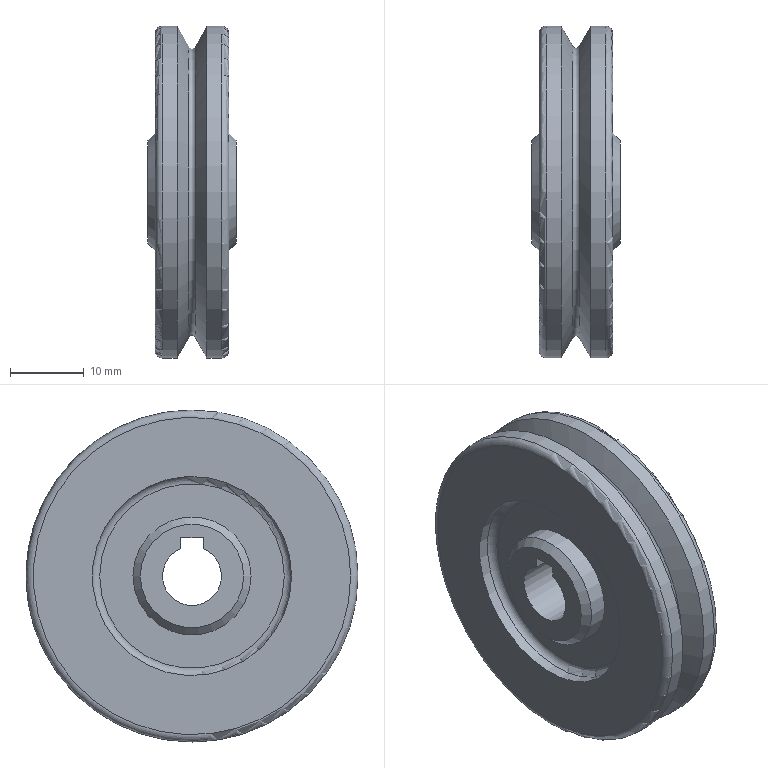Component | NX | ASSY_PRAC_PART_9 | 1 solid | 25 faces | volume 12810 mm3 | plane 9 | cylinder 7 | torus 5 | cone 4 | commonest cylinder face diameters 27 x2 16 x2 45 x2 8 x1